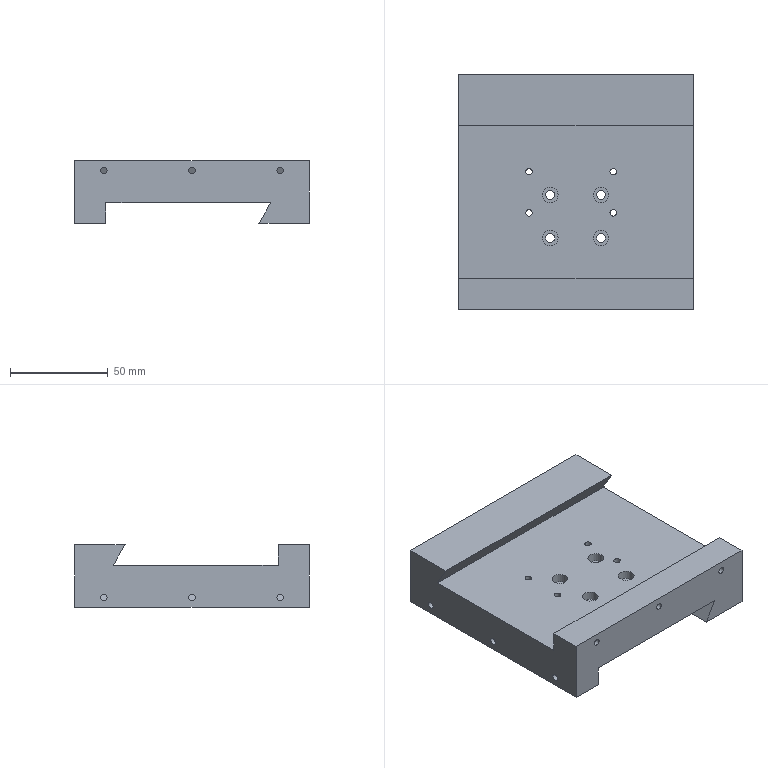Component | NX | SADDLE | 1 solid | 36 faces | volume 253582 mm3 | plane 18 | cylinder 18 | commonest cylinder face diameters 3.3 x10 4.5 x4 8 x4